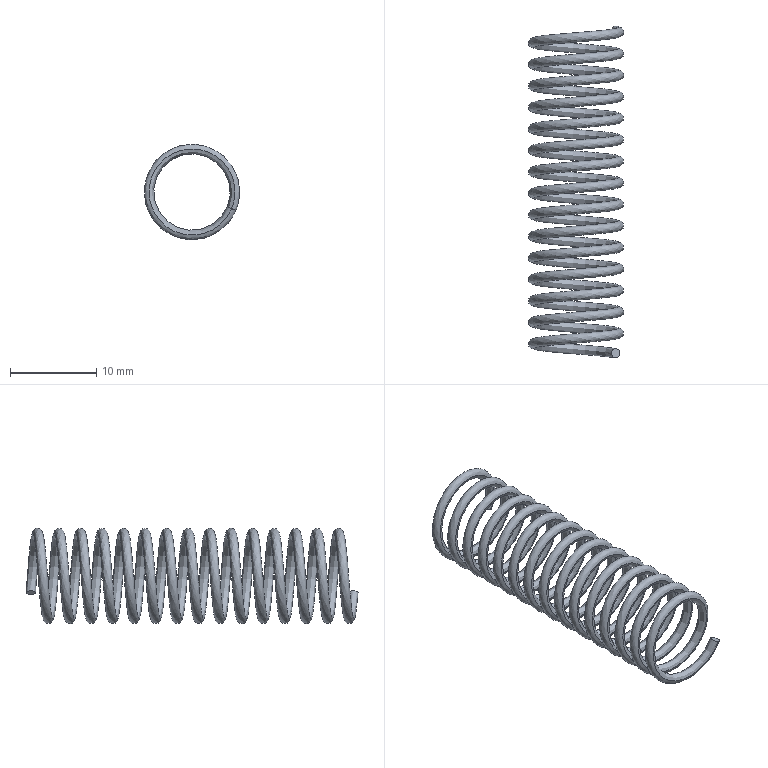Component | SolidWorks | Spring.1-1 | 1 solid | 4 faces | volume 447 mm3 | spline 2 | plane 2